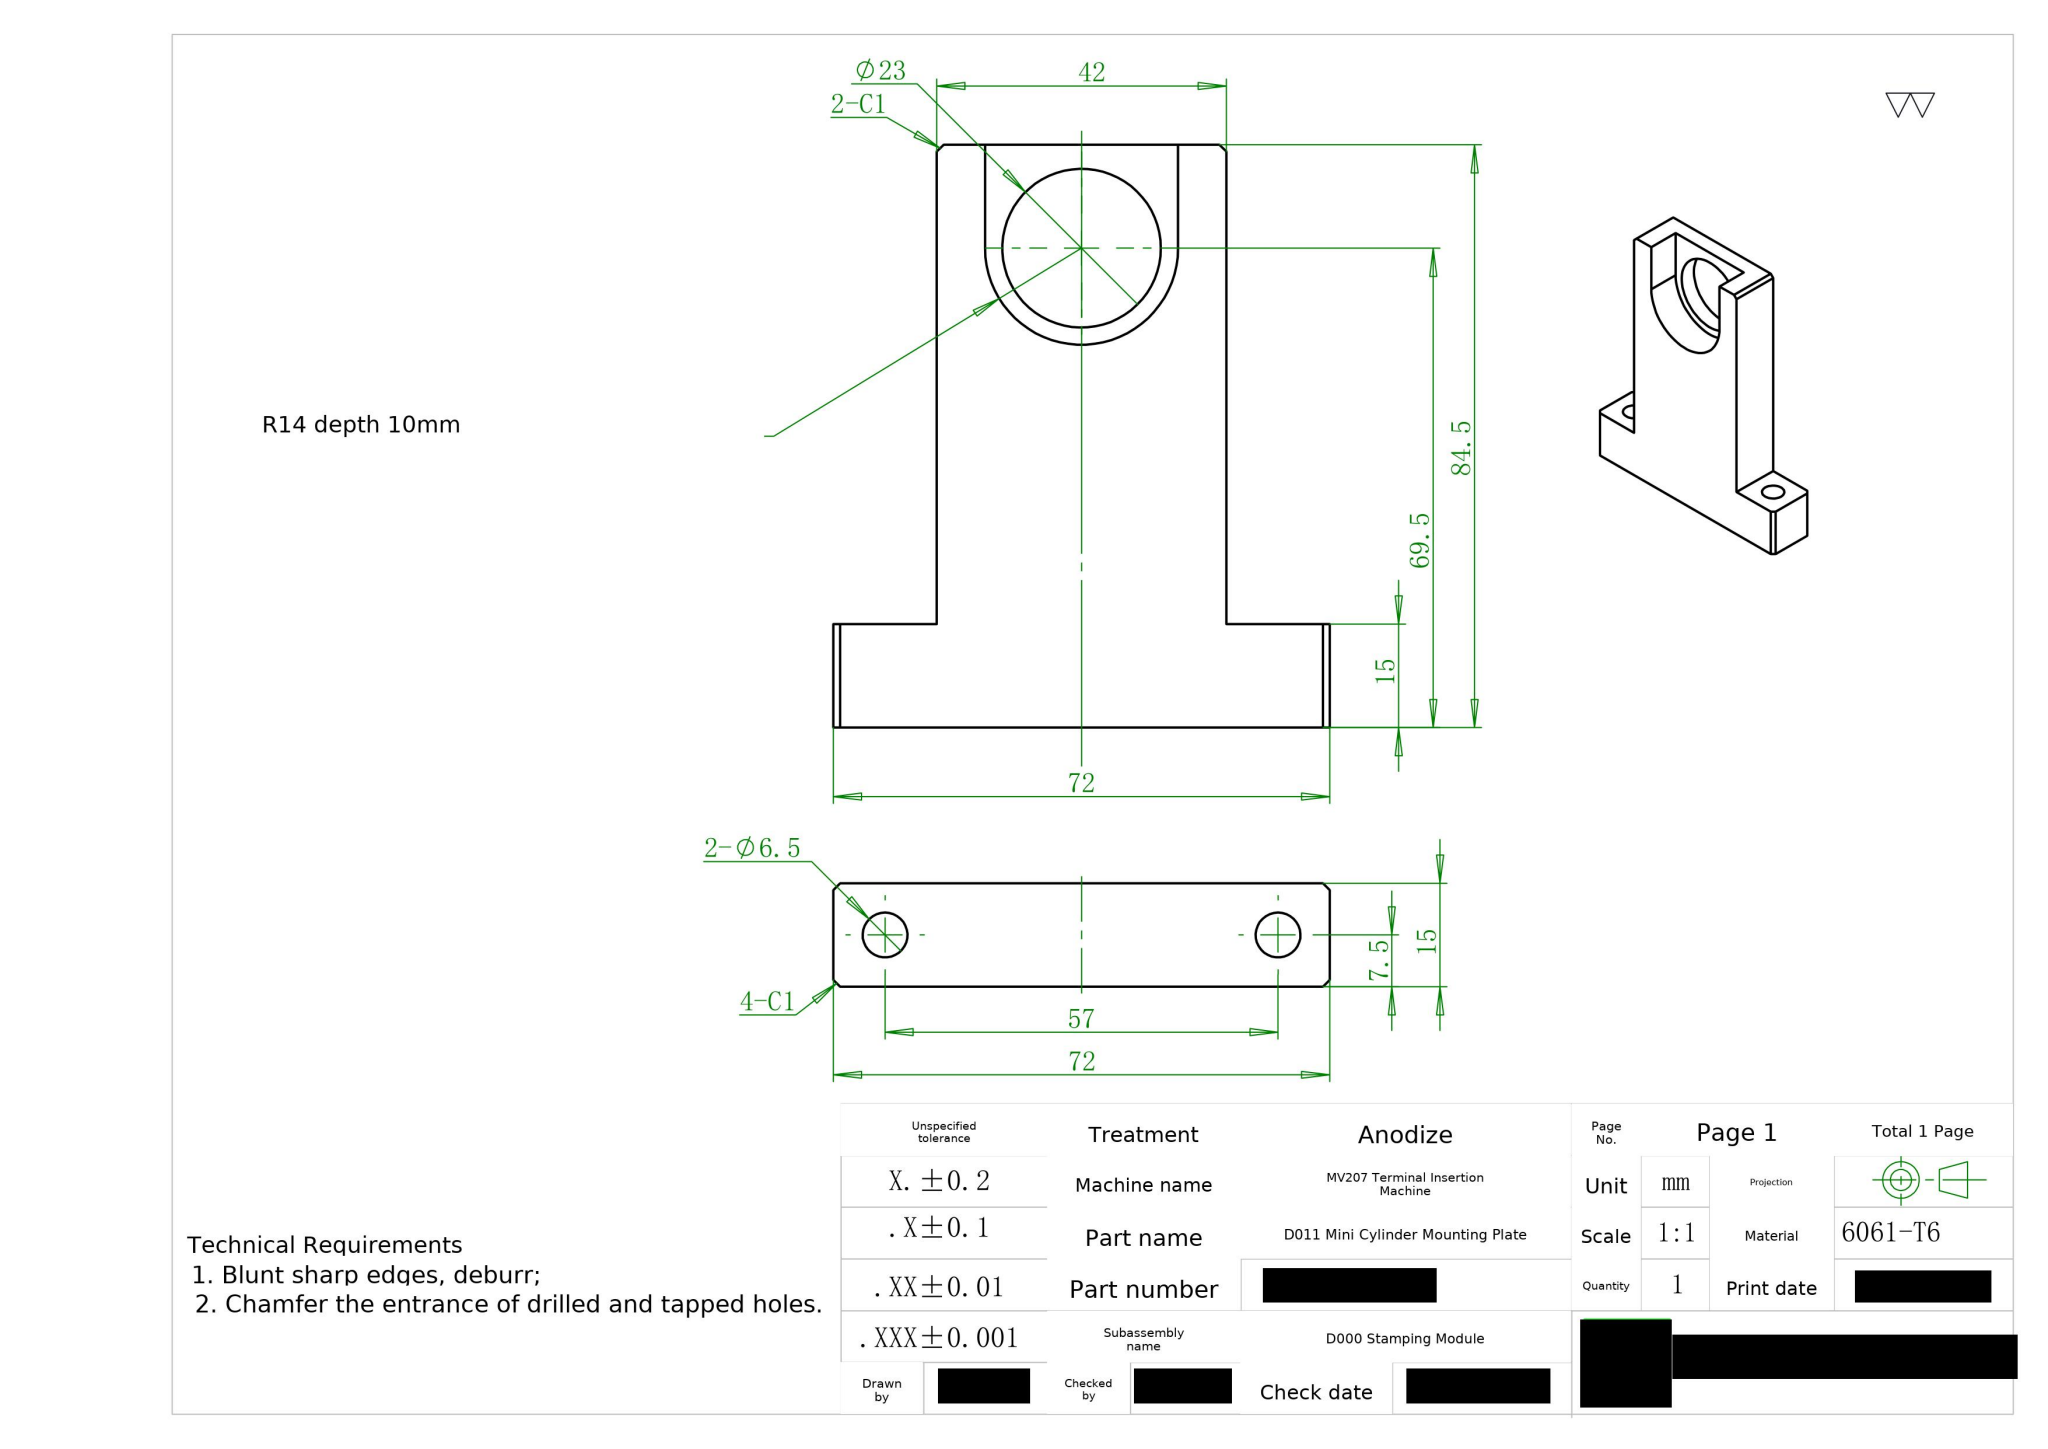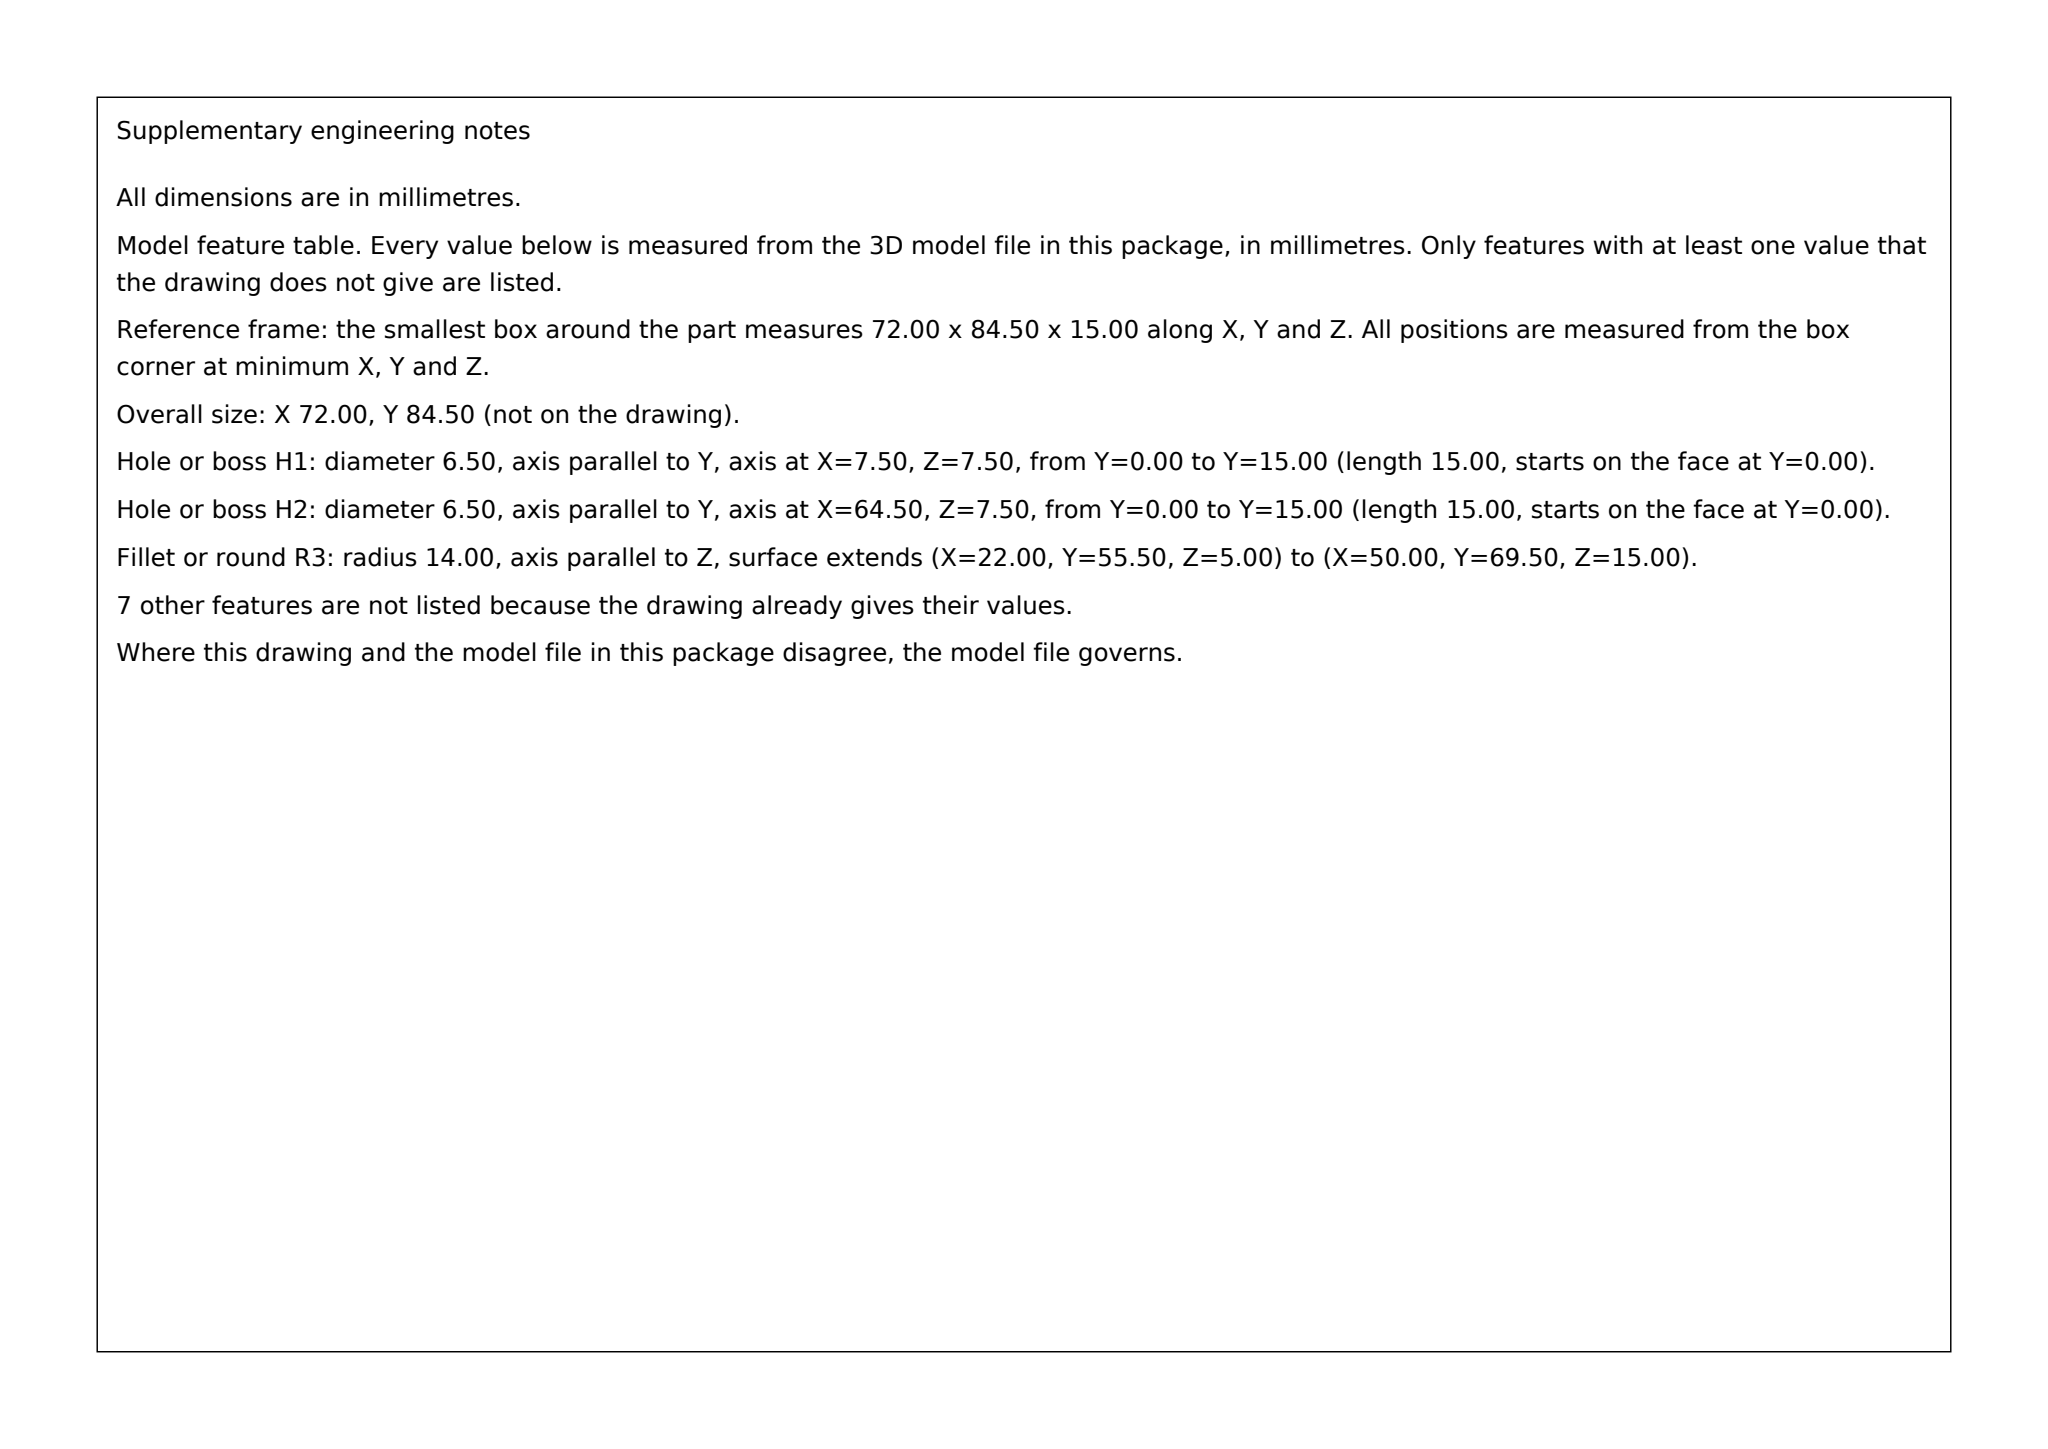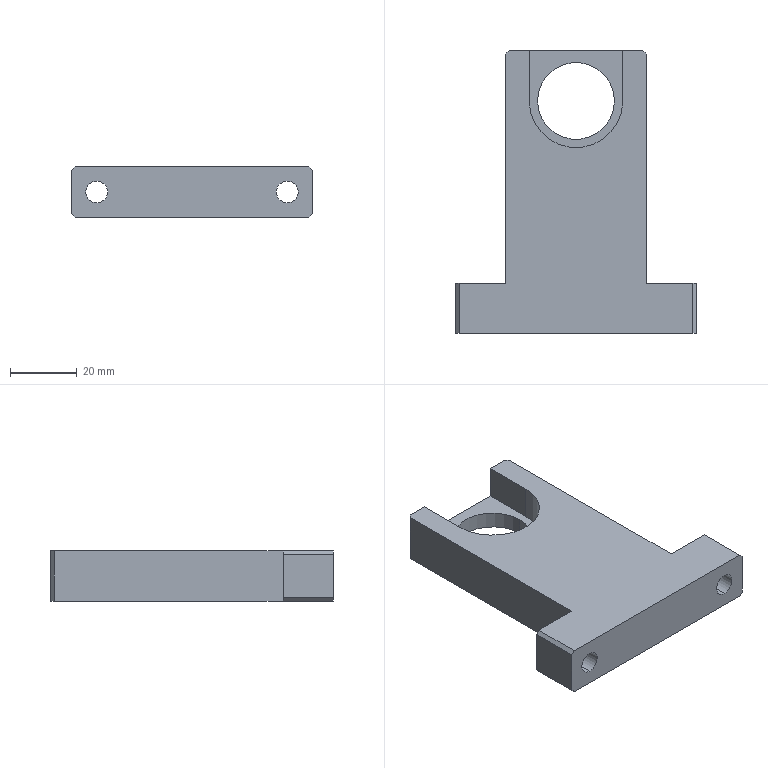Part | SolidWorks | mm | material 6061-T6 | 1 solid | 26 faces | box 72 x 84.5 x 15 mm | volume 49588 mm3 | plane 19 | cylinder 7 | commonest cylinder face diameters 6.5 x4 23 x2 28 x1
build123d program:
from build123d import *

# Parameters (mm, degrees)
SKETCH1_W                  = 42
SKETCH1_H                  = 15
BOSS_EXTRUDE1_DEPTH        = 84.5
SKETCH3_W                  = 15
SKETCH3_H                  = 15
BOSS_EXTRUDE2_DEPTH        = 15
SKETCH4_W                  = 15
SKETCH4_H                  = 15
BOSS_EXTRUDE3_DEPTH        = 15
F_6_5_6_5_DIAMETER_HOLE1_D = 6.5
CUT_EXTRUDE1_DEPTH         = 10
SKETCH11_R                 = 11.5
CUT_EXTRUDE2_DEPTH         = 93.392
CHAMFER1_SIZE              = 1


with BuildPart() as part:
    # Sketch1 → Boss-Extrude1 (new body)
    with BuildSketch(Plane(origin=(0, 0, 0), x_dir=(1, 0, 0), z_dir=(0, 1, 0))):
        Rectangle(SKETCH1_W, SKETCH1_H)
    extrude(amount=BOSS_EXTRUDE1_DEPTH)

    # Sketch3 → Boss-Extrude2 (add)
    with BuildSketch(Plane(origin=(21, 0, 0), x_dir=(0, 0, -1), z_dir=(1, 0, 0))):
        with Locations((0, 7.5)):
            Rectangle(SKETCH3_W, SKETCH3_H)
    extrude(amount=BOSS_EXTRUDE2_DEPTH)

    # Sketch4 → Boss-Extrude3 (add)
    with BuildSketch(Plane.ZY.offset(21)):
        with Locations((0, 7.5)):
            Rectangle(SKETCH4_W, SKETCH4_H)
    extrude(amount=BOSS_EXTRUDE3_DEPTH)

    # 6.5 _6.5_ Diameter Hole1 (through all)
    with Locations(Plane(origin=(0, 15, 0), x_dir=(1, 0, 0), z_dir=(0, 1, 0))):
        with Locations((-28.5, 0), (28.5, 0)):
            Hole(F_6_5_6_5_DIAMETER_HOLE1_D / 2)

    # Sketch10 → Cut-Extrude1 (cut)
    with BuildSketch(Plane.XY.offset(7.5)):
        with BuildLine():
            Line((14, 84.5), (14, 69.5))
            ThreePointArc((14, 69.5), (0, 55.5), (-14, 69.5))
            Line((-14, 69.5), (-14, 84.5))
            ThreePointArc((-14, 84.5), (0, 98.5), (14, 84.5))
        make_face()
    extrude(amount=-CUT_EXTRUDE1_DEPTH, mode=Mode.SUBTRACT)

    # Sketch11 → Cut-Extrude2 (cut, through all)
    with BuildSketch(Plane.XY.offset(-2.5)):
        with Locations((0, 69.5)):
            Circle(SKETCH11_R)
    extrude(amount=-CUT_EXTRUDE2_DEPTH, mode=Mode.SUBTRACT)

    # Chamfer1
    chamfer1_edges = [part.edges().sort_by_distance(p)[0] for p in [
        (-36, 7.5, 7.5),
        (-36, 7.5, -7.5),
        (36, 7.5, -7.5),
        (36, 7.5, 7.5),
        (21, 84.5, 0),
        (-21, 84.5, 0),
    ]]
    chamfer(chamfer1_edges, length=CHAMFER1_SIZE)


solid = part.part
STEP:
#1=CARTESIAN_POINT('',(-11.5,69.5,-7.5));
#2=VERTEX_POINT('',#1);
#3=CARTESIAN_POINT('',(11.5,69.5,-7.5));
#4=VERTEX_POINT('',#3);
#5=CARTESIAN_POINT('',(0.,69.5,-7.5));
#6=DIRECTION('',(0.,0.,1.));
#7=DIRECTION('',(1.,0.,0.));
#8=AXIS2_PLACEMENT_3D('',#5,#6,#7);
#9=CIRCLE('',#8,11.5);
#10=EDGE_CURVE('',#2,#4,#9,.T.);
#11=ORIENTED_EDGE('',*,*,#10,.F.);
#12=CARTESIAN_POINT('',(-11.5,69.5,-2.5));
#13=VERTEX_POINT('',#12);
#14=CARTESIAN_POINT('',(-11.5,69.5,-7.5));
#15=DIRECTION('',(0.,0.,1.));
#16=VECTOR('',#15,1000.);
#17=LINE('',#14,#16);
#18=EDGE_CURVE('',#2,#13,#17,.T.);
#19=ORIENTED_EDGE('',*,*,#18,.T.);
#20=CARTESIAN_POINT('',(11.5,69.5,-2.5));
#21=VERTEX_POINT('',#20);
#22=CARTESIAN_POINT('',(0.,69.5,-2.5));
#23=DIRECTION('',(0.,0.,1.));
#24=DIRECTION('',(1.,0.,0.));
#25=AXIS2_PLACEMENT_3D('',#22,#23,#24);
#26=CIRCLE('',#25,11.5);
#27=EDGE_CURVE('',#13,#21,#26,.T.);
#28=ORIENTED_EDGE('',*,*,#27,.T.);
#29=CARTESIAN_POINT('',(11.5,69.5,-7.5));
#30=DIRECTION('',(0.,0.,1.));
#31=VECTOR('',#30,1000.);
#32=LINE('',#29,#31);
#33=EDGE_CURVE('',#4,#21,#32,.T.);
#34=ORIENTED_EDGE('',*,*,#33,.F.);
#35=EDGE_LOOP('',(#11,#19,#28,#34));
#36=FACE_OUTER_BOUND('',#35,.T.);
#37=CARTESIAN_POINT('',(0.,69.5,-7.5));
#38=DIRECTION('',(0.,0.,1.));
#39=DIRECTION('',(1.,0.,0.));
#40=AXIS2_PLACEMENT_3D('',#37,#38,#39);
#41=CYLINDRICAL_SURFACE('',#40,11.5);
#42=ADVANCED_FACE('',(#36),#41,.F.);
#43=CARTESIAN_POINT('',(-28.5,0.,-3.25));
#44=VERTEX_POINT('',#43);
#45=CARTESIAN_POINT('',(-28.5,0.,3.25));
#46=VERTEX_POINT('',#45);
#47=CARTESIAN_POINT('',(-28.5,0.,0.));
#48=DIRECTION('',(0.,1.,0.));
#49=DIRECTION('',(0.,0.,1.));
#50=AXIS2_PLACEMENT_3D('',#47,#48,#49);
#51=CIRCLE('',#50,3.25);
#52=EDGE_CURVE('',#44,#46,#51,.T.);
#53=ORIENTED_EDGE('',*,*,#52,.F.);
#54=CARTESIAN_POINT('',(-28.5,15.,-3.25));
#55=VERTEX_POINT('',#54);
#56=CARTESIAN_POINT('',(-28.5,15.,-3.25));
#57=DIRECTION('',(0.,1.,0.));
#58=VECTOR('',#57,1000.);
#59=LINE('',#56,#58);
#60=EDGE_CURVE('',#44,#55,#59,.T.);
#61=ORIENTED_EDGE('',*,*,#60,.T.);
#62=CARTESIAN_POINT('',(-28.5,15.,3.25));
#63=VERTEX_POINT('',#62);
#64=CARTESIAN_POINT('',(-28.5,15.,0.));
#65=DIRECTION('',(0.,1.,0.));
#66=DIRECTION('',(0.,0.,1.));
#67=AXIS2_PLACEMENT_3D('',#64,#65,#66);
#68=CIRCLE('',#67,3.25);
#69=EDGE_CURVE('',#55,#63,#68,.T.);
#70=ORIENTED_EDGE('',*,*,#69,.T.);
#71=CARTESIAN_POINT('',(-28.5,15.,3.25));
#72=DIRECTION('',(0.,1.,0.));
#73=VECTOR('',#72,1000.);
#74=LINE('',#71,#73);
#75=EDGE_CURVE('',#46,#63,#74,.T.);
#76=ORIENTED_EDGE('',*,*,#75,.F.);
#77=EDGE_LOOP('',(#53,#61,#70,#76));
#78=FACE_OUTER_BOUND('',#77,.T.);
#79=CARTESIAN_POINT('',(-28.5,15.,0.));
#80=DIRECTION('',(0.,1.,0.));
#81=DIRECTION('',(0.,0.,1.));
#82=AXIS2_PLACEMENT_3D('',#79,#80,#81);
#83=CYLINDRICAL_SURFACE('',#82,3.25);
#84=ADVANCED_FACE('',(#78),#83,.F.);
#85=CARTESIAN_POINT('',(28.5,0.,-3.25));
#86=VERTEX_POINT('',#85);
#87=CARTESIAN_POINT('',(28.5,0.,3.25));
#88=VERTEX_POINT('',#87);
#89=CARTESIAN_POINT('',(28.5,0.,0.));
#90=DIRECTION('',(0.,1.,0.));
#91=DIRECTION('',(0.,0.,1.));
#92=AXIS2_PLACEMENT_3D('',#89,#90,#91);
#93=CIRCLE('',#92,3.25);
#94=EDGE_CURVE('',#86,#88,#93,.T.);
#95=ORIENTED_EDGE('',*,*,#94,.F.);
#96=CARTESIAN_POINT('',(28.5,15.,-3.25));
#97=VERTEX_POINT('',#96);
#98=CARTESIAN_POINT('',(28.5,15.,-3.25));
#99=DIRECTION('',(0.,1.,0.));
#100=VECTOR('',#99,1000.);
#101=LINE('',#98,#100);
#102=EDGE_CURVE('',#86,#97,#101,.T.);
#103=ORIENTED_EDGE('',*,*,#102,.T.);
#104=CARTESIAN_POINT('',(28.5,15.,3.25));
#105=VERTEX_POINT('',#104);
#106=CARTESIAN_POINT('',(28.5,15.,0.));
#107=DIRECTION('',(0.,1.,0.));
#108=DIRECTION('',(0.,0.,1.));
#109=AXIS2_PLACEMENT_3D('',#106,#107,#108);
#110=CIRCLE('',#109,3.25);
#111=EDGE_CURVE('',#97,#105,#110,.T.);
#112=ORIENTED_EDGE('',*,*,#111,.T.);
#113=CARTESIAN_POINT('',(28.5,15.,3.25));
#114=DIRECTION('',(0.,1.,0.));
#115=VECTOR('',#114,1000.);
#116=LINE('',#113,#115);
#117=EDGE_CURVE('',#88,#105,#116,.T.);
#118=ORIENTED_EDGE('',*,*,#117,.F.);
#119=EDGE_LOOP('',(#95,#103,#112,#118));
#120=FACE_OUTER_BOUND('',#119,.T.);
#121=CARTESIAN_POINT('',(28.5,15.,0.));
#122=DIRECTION('',(0.,1.,0.));
#123=DIRECTION('',(0.,0.,1.));
#124=AXIS2_PLACEMENT_3D('',#121,#122,#123);
#125=CYLINDRICAL_SURFACE('',#124,3.25);
#126=ADVANCED_FACE('',(#120),#125,.F.);
#127=CARTESIAN_POINT('',(-21.,83.5,7.5));
#128=VERTEX_POINT('',#127);
#129=CARTESIAN_POINT('',(-21.,15.,7.5));
#130=VERTEX_POINT('',#129);
#131=CARTESIAN_POINT('',(-21.,84.5,7.5));
#132=DIRECTION('',(0.,-1.,0.));
#133=VECTOR('',#132,1000.);
#134=LINE('',#131,#133);
#135=EDGE_CURVE('',#128,#130,#134,.T.);
#136=ORIENTED_EDGE('',*,*,#135,.F.);
#137=CARTESIAN_POINT('',(-21.,83.5,-7.5));
#138=VERTEX_POINT('',#137);
#139=CARTESIAN_POINT('',(-21.,83.5,-7.5));
#140=DIRECTION('',(0.,0.,-1.));
#141=VECTOR('',#140,1000.);
#142=LINE('',#139,#141);
#143=EDGE_CURVE('',#128,#138,#142,.T.);
#144=ORIENTED_EDGE('',*,*,#143,.T.);
#145=CARTESIAN_POINT('',(-21.,15.,-7.5));
#146=VERTEX_POINT('',#145);
#147=CARTESIAN_POINT('',(-21.,84.5,-7.5));
#148=DIRECTION('',(0.,-1.,0.));
#149=VECTOR('',#148,1000.);
#150=LINE('',#147,#149);
#151=EDGE_CURVE('',#138,#146,#150,.T.);
#152=ORIENTED_EDGE('',*,*,#151,.T.);
#153=CARTESIAN_POINT('',(-21.,15.,7.5));
#154=DIRECTION('',(0.,-0.,-1.));
#155=VECTOR('',#154,1000.);
#156=LINE('',#153,#155);
#157=EDGE_CURVE('',#130,#146,#156,.T.);
#158=ORIENTED_EDGE('',*,*,#157,.F.);
#159=EDGE_LOOP('',(#136,#144,#152,#158));
#160=FACE_OUTER_BOUND('',#159,.T.);
#161=CARTESIAN_POINT('',(-21.,84.5,-7.5));
#162=DIRECTION('',(1.,0.,0.));
#163=DIRECTION('',(0.,0.,-1.));
#164=AXIS2_PLACEMENT_3D('',#161,#162,#163);
#165=PLANE('',#164);
#166=ADVANCED_FACE('',(#160),#165,.F.);
#167=CARTESIAN_POINT('',(21.,83.5,-7.5));
#168=VERTEX_POINT('',#167);
#169=CARTESIAN_POINT('',(21.,15.,-7.5));
#170=VERTEX_POINT('',#169);
#171=CARTESIAN_POINT('',(21.,84.5,-7.5));
#172=DIRECTION('',(0.,-1.,0.));
#173=VECTOR('',#172,1000.);
#174=LINE('',#171,#173);
#175=EDGE_CURVE('',#168,#170,#174,.T.);
#176=ORIENTED_EDGE('',*,*,#175,.F.);
#177=CARTESIAN_POINT('',(21.,83.5,7.5));
#178=VERTEX_POINT('',#177);
#179=CARTESIAN_POINT('',(21.,83.5,7.5));
#180=DIRECTION('',(0.,0.,1.));
#181=VECTOR('',#180,1000.);
#182=LINE('',#179,#181);
#183=EDGE_CURVE('',#168,#178,#182,.T.);
#184=ORIENTED_EDGE('',*,*,#183,.T.);
#185=CARTESIAN_POINT('',(21.,15.,7.5));
#186=VERTEX_POINT('',#185);
#187=CARTESIAN_POINT('',(21.,84.5,7.5));
#188=DIRECTION('',(0.,-1.,0.));
#189=VECTOR('',#188,1000.);
#190=LINE('',#187,#189);
#191=EDGE_CURVE('',#178,#186,#190,.T.);
#192=ORIENTED_EDGE('',*,*,#191,.T.);
#193=CARTESIAN_POINT('',(21.,15.,7.5));
#194=DIRECTION('',(0.,0.,1.));
#195=VECTOR('',#194,1000.);
#196=LINE('',#193,#195);
#197=EDGE_CURVE('',#170,#186,#196,.T.);
#198=ORIENTED_EDGE('',*,*,#197,.F.);
#199=EDGE_LOOP('',(#176,#184,#192,#198));
#200=FACE_OUTER_BOUND('',#199,.T.);
#201=CARTESIAN_POINT('',(21.,84.5,-7.5));
#202=DIRECTION('',(-1.,0.,0.));
#203=DIRECTION('',(0.,0.,1.));
#204=AXIS2_PLACEMENT_3D('',#201,#202,#203);
#205=PLANE('',#204);
#206=ADVANCED_FACE('',(#200),#205,.F.);
#207=CARTESIAN_POINT('',(0.,69.5,-7.5));
#208=DIRECTION('',(0.,0.,1.));
#209=DIRECTION('',(1.,0.,0.));
#210=AXIS2_PLACEMENT_3D('',#207,#208,#209);
#211=CIRCLE('',#210,11.5);
#212=EDGE_CURVE('',#4,#2,#211,.T.);
#213=ORIENTED_EDGE('',*,*,#212,.T.);
#214=ORIENTED_EDGE('',*,*,#10,.T.);
#215=EDGE_LOOP('',(#213,#214));
#216=FACE_BOUND('',#215,.T.);
#217=CARTESIAN_POINT('',(35.,0.,-7.5));
#218=VERTEX_POINT('',#217);
#219=CARTESIAN_POINT('',(-35.,0.,-7.5));
#220=VERTEX_POINT('',#219);
#221=CARTESIAN_POINT('',(-21.,0.,-7.5));
#222=DIRECTION('',(-1.,0.,0.));
#223=VECTOR('',#222,1000.);
#224=LINE('',#221,#223);
#225=EDGE_CURVE('',#218,#220,#224,.T.);
#226=ORIENTED_EDGE('',*,*,#225,.T.);
#227=CARTESIAN_POINT('',(-35.,15.,-7.5));
#228=VERTEX_POINT('',#227);
#229=CARTESIAN_POINT('',(-35.,15.,-7.5));
#230=DIRECTION('',(0.,1.,0.));
#231=VECTOR('',#230,1000.);
#232=LINE('',#229,#231);
#233=EDGE_CURVE('',#220,#228,#232,.T.);
#234=ORIENTED_EDGE('',*,*,#233,.T.);
#235=CARTESIAN_POINT('',(-36.,15.,-7.5));
#236=DIRECTION('',(1.,0.,0.));
#237=VECTOR('',#236,1000.);
#238=LINE('',#235,#237);
#239=EDGE_CURVE('',#228,#146,#238,.T.);
#240=ORIENTED_EDGE('',*,*,#239,.T.);
#241=ORIENTED_EDGE('',*,*,#151,.F.);
#242=CARTESIAN_POINT('',(-20.,84.5,-7.5));
#243=VERTEX_POINT('',#242);
#244=CARTESIAN_POINT('',(-20.,84.5,-7.5));
#245=DIRECTION('',(0.7071,0.7071,0.));
#246=VECTOR('',#245,1000.);
#247=LINE('',#244,#246);
#248=EDGE_CURVE('',#138,#243,#247,.T.);
#249=ORIENTED_EDGE('',*,*,#248,.T.);
#250=CARTESIAN_POINT('',(20.,84.5,-7.5));
#251=VERTEX_POINT('',#250);
#252=CARTESIAN_POINT('',(-21.,84.5,-7.5));
#253=DIRECTION('',(-1.,0.,0.));
#254=VECTOR('',#253,1000.);
#255=LINE('',#252,#254);
#256=EDGE_CURVE('',#251,#243,#255,.T.);
#257=ORIENTED_EDGE('',*,*,#256,.F.);
#258=CARTESIAN_POINT('',(20.,84.5,-7.5));
#259=DIRECTION('',(0.7071,-0.7071,0.));
#260=VECTOR('',#259,1000.);
#261=LINE('',#258,#260);
#262=EDGE_CURVE('',#251,#168,#261,.T.);
#263=ORIENTED_EDGE('',*,*,#262,.T.);
#264=ORIENTED_EDGE('',*,*,#175,.T.);
#265=CARTESIAN_POINT('',(35.,15.,-7.5));
#266=VERTEX_POINT('',#265);
#267=CARTESIAN_POINT('',(36.,15.,-7.5));
#268=DIRECTION('',(-1.,0.,0.));
#269=VECTOR('',#268,1000.);
#270=LINE('',#267,#269);
#271=EDGE_CURVE('',#266,#170,#270,.T.);
#272=ORIENTED_EDGE('',*,*,#271,.F.);
#273=CARTESIAN_POINT('',(35.,84.5,-7.5));
#274=DIRECTION('',(0.,-1.,0.));
#275=VECTOR('',#274,1000.);
#276=LINE('',#273,#275);
#277=EDGE_CURVE('',#266,#218,#276,.T.);
#278=ORIENTED_EDGE('',*,*,#277,.T.);
#279=EDGE_LOOP('',(#226,#234,#240,#241,#249,#257,#263,#264,#272,#278));
#280=FACE_OUTER_BOUND('',#279,.T.);
#281=CARTESIAN_POINT('',(-21.,84.5,-7.5));
#282=DIRECTION('',(0.,0.,1.));
#283=DIRECTION('',(1.,0.,0.));
#284=AXIS2_PLACEMENT_3D('',#281,#282,#283);
#285=PLANE('',#284);
#286=ADVANCED_FACE('',(#216,#280),#285,.F.);
#287=CARTESIAN_POINT('',(-35.,15.,7.5));
#288=VERTEX_POINT('',#287);
#289=CARTESIAN_POINT('',(-36.,15.,7.5));
#290=DIRECTION('',(1.,0.,0.));
#291=VECTOR('',#290,1000.);
#292=LINE('',#289,#291);
#293=EDGE_CURVE('',#288,#130,#292,.T.);
#294=ORIENTED_EDGE('',*,*,#293,.F.);
#295=CARTESIAN_POINT('',(-35.,0.,7.5));
#296=VERTEX_POINT('',#295);
#297=CARTESIAN_POINT('',(-35.,0.,7.5));
#298=DIRECTION('',(0.,-1.,0.));
#299=VECTOR('',#298,1000.);
#300=LINE('',#297,#299);
#301=EDGE_CURVE('',#288,#296,#300,.T.);
#302=ORIENTED_EDGE('',*,*,#301,.T.);
#303=CARTESIAN_POINT('',(35.,0.,7.5));
#304=VERTEX_POINT('',#303);
#305=CARTESIAN_POINT('',(-21.,0.,7.5));
#306=DIRECTION('',(1.,0.,0.));
#307=VECTOR('',#306,1000.);
#308=LINE('',#305,#307);
#309=EDGE_CURVE('',#296,#304,#308,.T.);
#310=ORIENTED_EDGE('',*,*,#309,.T.);
#311=CARTESIAN_POINT('',(35.,15.,7.5));
#312=VERTEX_POINT('',#311);
#313=CARTESIAN_POINT('',(35.,84.5,7.5));
#314=DIRECTION('',(0.,1.,0.));
#315=VECTOR('',#314,1000.);
#316=LINE('',#313,#315);
#317=EDGE_CURVE('',#304,#312,#316,.T.);
#318=ORIENTED_EDGE('',*,*,#317,.T.);
#319=CARTESIAN_POINT('',(36.,15.,7.5));
#320=DIRECTION('',(-1.,0.,0.));
#321=VECTOR('',#320,1000.);
#322=LINE('',#319,#321);
#323=EDGE_CURVE('',#312,#186,#322,.T.);
#324=ORIENTED_EDGE('',*,*,#323,.T.);
#325=ORIENTED_EDGE('',*,*,#191,.F.);
#326=CARTESIAN_POINT('',(20.,84.5,7.5));
#327=VERTEX_POINT('',#326);
#328=CARTESIAN_POINT('',(20.,84.5,7.5));
#329=DIRECTION('',(-0.7071,0.7071,0.));
#330=VECTOR('',#329,1000.);
#331=LINE('',#328,#330);
#332=EDGE_CURVE('',#178,#327,#331,.T.);
#333=ORIENTED_EDGE('',*,*,#332,.T.);
#334=CARTESIAN_POINT('',(14.,84.5,7.5));
#335=VERTEX_POINT('',#334);
#336=CARTESIAN_POINT('',(-21.,84.5,7.5));
#337=DIRECTION('',(1.,0.,0.));
#338=VECTOR('',#337,1000.);
#339=LINE('',#336,#338);
#340=EDGE_CURVE('',#335,#327,#339,.T.);
#341=ORIENTED_EDGE('',*,*,#340,.F.);
#342=CARTESIAN_POINT('',(14.,69.5,7.5));
#343=VERTEX_POINT('',#342);
#344=CARTESIAN_POINT('',(14.,84.5,7.5));
#345=DIRECTION('',(0.,1.,0.));
#346=VECTOR('',#345,1000.);
#347=LINE('',#344,#346);
#348=EDGE_CURVE('',#343,#335,#347,.T.);
#349=ORIENTED_EDGE('',*,*,#348,.F.);
#350=CARTESIAN_POINT('',(-14.,69.5,7.5));
#351=VERTEX_POINT('',#350);
#352=CARTESIAN_POINT('',(0.,69.5,7.5));
#353=DIRECTION('',(0.,0.,1.));
#354=DIRECTION('',(1.,0.,0.));
#355=AXIS2_PLACEMENT_3D('',#352,#353,#354);
#356=CIRCLE('',#355,14.);
#357=EDGE_CURVE('',#351,#343,#356,.T.);
#358=ORIENTED_EDGE('',*,*,#357,.F.);
#359=CARTESIAN_POINT('',(-14.,84.5,7.5));
#360=VERTEX_POINT('',#359);
#361=CARTESIAN_POINT('',(-14.,84.5,7.5));
#362=DIRECTION('',(0.,-1.,0.));
#363=VECTOR('',#362,1000.);
#364=LINE('',#361,#363);
#365=EDGE_CURVE('',#360,#351,#364,.T.);
#366=ORIENTED_EDGE('',*,*,#365,.F.);
#367=CARTESIAN_POINT('',(-20.,84.5,7.5));
#368=VERTEX_POINT('',#367);
#369=CARTESIAN_POINT('',(-21.,84.5,7.5));
#370=DIRECTION('',(1.,0.,0.));
#371=VECTOR('',#370,1000.);
#372=LINE('',#369,#371);
#373=EDGE_CURVE('',#368,#360,#372,.T.);
#374=ORIENTED_EDGE('',*,*,#373,.F.);
#375=CARTESIAN_POINT('',(-20.,84.5,7.5));
#376=DIRECTION('',(-0.7071,-0.7071,0.));
#377=VECTOR('',#376,1000.);
#378=LINE('',#375,#377);
#379=EDGE_CURVE('',#368,#128,#378,.T.);
#380=ORIENTED_EDGE('',*,*,#379,.T.);
#381=ORIENTED_EDGE('',*,*,#135,.T.);
#382=EDGE_LOOP('',(#294,#302,#310,#318,#324,#325,#333,#341,#349,#358,#366,#374,#380,#381));
#383=FACE_OUTER_BOUND('',#382,.T.);
#384=CARTESIAN_POINT('',(-21.,84.5,7.5));
#385=DIRECTION('',(0.,0.,-1.));
#386=DIRECTION('',(-1.,0.,0.));
#387=AXIS2_PLACEMENT_3D('',#384,#385,#386);
#388=PLANE('',#387);
#389=ADVANCED_FACE('',(#383),#388,.F.);
#390=ORIENTED_EDGE('',*,*,#340,.T.);
#391=CARTESIAN_POINT('',(20.,84.5,-7.5));
#392=DIRECTION('',(0.,0.,-1.));
#393=VECTOR('',#392,1000.);
#394=LINE('',#391,#393);
#395=EDGE_CURVE('',#327,#251,#394,.T.);
#396=ORIENTED_EDGE('',*,*,#395,.T.);
#397=ORIENTED_EDGE('',*,*,#256,.T.);
#398=CARTESIAN_POINT('',(-20.,84.5,7.5));
#399=DIRECTION('',(0.,0.,1.));
#400=VECTOR('',#399,1000.);
#401=LINE('',#398,#400);
#402=EDGE_CURVE('',#243,#368,#401,.T.);
#403=ORIENTED_EDGE('',*,*,#402,.T.);
#404=ORIENTED_EDGE('',*,*,#373,.T.);
#405=CARTESIAN_POINT('',(-14.,84.5,-2.5));
#406=VERTEX_POINT('',#405);
#407=CARTESIAN_POINT('',(-14.,84.5,-2.5));
#408=DIRECTION('',(0.,0.,1.));
#409=VECTOR('',#408,1000.);
#410=LINE('',#407,#409);
#411=EDGE_CURVE('',#406,#360,#410,.T.);
#412=ORIENTED_EDGE('',*,*,#411,.F.);
#413=CARTESIAN_POINT('',(14.,84.5,-2.5));
#414=VERTEX_POINT('',#413);
#415=CARTESIAN_POINT('',(0.,84.5,-2.5));
#416=DIRECTION('',(1.,0.,0.));
#417=VECTOR('',#416,1000.);
#418=LINE('',#415,#417);
#419=EDGE_CURVE('',#406,#414,#418,.T.);
#420=ORIENTED_EDGE('',*,*,#419,.T.);
#421=CARTESIAN_POINT('',(14.,84.5,-2.5));
#422=DIRECTION('',(0.,0.,1.));
#423=VECTOR('',#422,1000.);
#424=LINE('',#421,#423);
#425=EDGE_CURVE('',#414,#335,#424,.T.);
#426=ORIENTED_EDGE('',*,*,#425,.T.);
#427=EDGE_LOOP('',(#390,#396,#397,#403,#404,#412,#420,#426));
#428=FACE_OUTER_BOUND('',#427,.T.);
#429=CARTESIAN_POINT('',(0.,84.5,0.));
#430=DIRECTION('',(0.,1.,0.));
#431=DIRECTION('',(0.,0.,1.));
#432=AXIS2_PLACEMENT_3D('',#429,#430,#431);
#433=PLANE('',#432);
#434=ADVANCED_FACE('',(#428),#433,.T.);
#435=CARTESIAN_POINT('',(-28.5,0.,0.));
#436=DIRECTION('',(0.,1.,0.));
#437=DIRECTION('',(0.,0.,1.));
#438=AXIS2_PLACEMENT_3D('',#435,#436,#437);
#439=CIRCLE('',#438,3.25);
#440=EDGE_CURVE('',#46,#44,#439,.T.);
#441=ORIENTED_EDGE('',*,*,#440,.T.);
#442=ORIENTED_EDGE('',*,*,#52,.T.);
#443=EDGE_LOOP('',(#441,#442));
#444=FACE_BOUND('',#443,.T.);
#445=CARTESIAN_POINT('',(28.5,0.,0.));
#446=DIRECTION('',(0.,1.,0.));
#447=DIRECTION('',(0.,0.,1.));
#448=AXIS2_PLACEMENT_3D('',#445,#446,#447);
#449=CIRCLE('',#448,3.25);
#450=EDGE_CURVE('',#88,#86,#449,.T.);
#451=ORIENTED_EDGE('',*,*,#450,.T.);
#452=ORIENTED_EDGE('',*,*,#94,.T.);
#453=EDGE_LOOP('',(#451,#452));
#454=FACE_BOUND('',#453,.T.);
#455=ORIENTED_EDGE('',*,*,#309,.F.);
#456=CARTESIAN_POINT('',(-36.,-0.,6.5));
#457=VERTEX_POINT('',#456);
#458=CARTESIAN_POINT('',(-36.,0.,6.5));
#459=DIRECTION('',(-0.7071,0.,-0.7071));
#460=VECTOR('',#459,1000.);
#461=LINE('',#458,#460);
#462=EDGE_CURVE('',#296,#457,#461,.T.);
#463=ORIENTED_EDGE('',*,*,#462,.T.);
#464=CARTESIAN_POINT('',(-36.,-0.,-6.5));
#465=VERTEX_POINT('',#464);
#466=CARTESIAN_POINT('',(-36.,0.,7.5));
#467=DIRECTION('',(0.,0.,1.));
#468=VECTOR('',#467,1000.);
#469=LINE('',#466,#468);
#470=EDGE_CURVE('',#465,#457,#469,.T.);
#471=ORIENTED_EDGE('',*,*,#470,.F.);
#472=CARTESIAN_POINT('',(-36.,0.,-6.5));
#473=DIRECTION('',(0.7071,0.,-0.7071));
#474=VECTOR('',#473,1000.);
#475=LINE('',#472,#474);
#476=EDGE_CURVE('',#465,#220,#475,.T.);
#477=ORIENTED_EDGE('',*,*,#476,.T.);
#478=ORIENTED_EDGE('',*,*,#225,.F.);
#479=CARTESIAN_POINT('',(36.,0.,-6.5));
#480=VERTEX_POINT('',#479);
#481=CARTESIAN_POINT('',(36.,0.,-6.5));
#482=DIRECTION('',(0.7071,0.,0.7071));
#483=VECTOR('',#482,1000.);
#484=LINE('',#481,#483);
#485=EDGE_CURVE('',#218,#480,#484,.T.);
#486=ORIENTED_EDGE('',*,*,#485,.T.);
#487=CARTESIAN_POINT('',(36.,0.,6.5));
#488=VERTEX_POINT('',#487);
#489=CARTESIAN_POINT('',(36.,0.,7.5));
#490=DIRECTION('',(0.,0.,-1.));
#491=VECTOR('',#490,1000.);
#492=LINE('',#489,#491);
#493=EDGE_CURVE('',#488,#480,#492,.T.);
#494=ORIENTED_EDGE('',*,*,#493,.F.);
#495=CARTESIAN_POINT('',(36.,0.,6.5));
#496=DIRECTION('',(-0.7071,0.,0.7071));
#497=VECTOR('',#496,1000.);
#498=LINE('',#495,#497);
#499=EDGE_CURVE('',#488,#304,#498,.T.);
#500=ORIENTED_EDGE('',*,*,#499,.T.);
#501=EDGE_LOOP('',(#455,#463,#471,#477,#478,#486,#494,#500));
#502=FACE_OUTER_BOUND('',#501,.T.);
#503=CARTESIAN_POINT('',(0.,0.,0.));
#504=DIRECTION('',(0.,1.,0.));
#505=DIRECTION('',(0.,0.,1.));
#506=AXIS2_PLACEMENT_3D('',#503,#504,#505);
#507=PLANE('',#506);
#508=ADVANCED_FACE('',(#444,#454,#502),#507,.F.);
#509=CARTESIAN_POINT('',(28.5,15.,0.));
#510=DIRECTION('',(0.,1.,0.));
#511=DIRECTION('',(0.,0.,1.));
#512=AXIS2_PLACEMENT_3D('',#509,#510,#511);
#513=CIRCLE('',#512,3.25);
#514=EDGE_CURVE('',#105,#97,#513,.T.);
#515=ORIENTED_EDGE('',*,*,#514,.F.);
#516=ORIENTED_EDGE('',*,*,#111,.F.);
#517=EDGE_LOOP('',(#515,#516));
#518=FACE_BOUND('',#517,.T.);
#519=CARTESIAN_POINT('',(36.,15.,-6.5));
#520=VERTEX_POINT('',#519);
#521=CARTESIAN_POINT('',(36.,15.,6.5));
#522=VERTEX_POINT('',#521);
#523=CARTESIAN_POINT('',(36.,15.,7.5));
#524=DIRECTION('',(0.,0.,1.));
#525=VECTOR('',#524,1000.);
#526=LINE('',#523,#525);
#527=EDGE_CURVE('',#520,#522,#526,.T.);
#528=ORIENTED_EDGE('',*,*,#527,.F.);
#529=CARTESIAN_POINT('',(36.,15.,-6.5));
#530=DIRECTION('',(-0.7071,0.,-0.7071));
#531=VECTOR('',#530,1000.);
#532=LINE('',#529,#531);
#533=EDGE_CURVE('',#520,#266,#532,.T.);
#534=ORIENTED_EDGE('',*,*,#533,.T.);
#535=ORIENTED_EDGE('',*,*,#271,.T.);
#536=ORIENTED_EDGE('',*,*,#197,.T.);
#537=ORIENTED_EDGE('',*,*,#323,.F.);
#538=CARTESIAN_POINT('',(36.,15.,6.5));
#539=DIRECTION('',(0.7071,0.,-0.7071));
#540=VECTOR('',#539,1000.);
#541=LINE('',#538,#540);
#542=EDGE_CURVE('',#312,#522,#541,.T.);
#543=ORIENTED_EDGE('',*,*,#542,.T.);
#544=EDGE_LOOP('',(#528,#534,#535,#536,#537,#543));
#545=FACE_OUTER_BOUND('',#544,.T.);
#546=CARTESIAN_POINT('',(36.,15.,7.5));
#547=DIRECTION('',(0.,-1.,0.));
#548=DIRECTION('',(0.,0.,-1.));
#549=AXIS2_PLACEMENT_3D('',#546,#547,#548);
#550=PLANE('',#549);
#551=ADVANCED_FACE('',(#518,#545),#550,.F.);
#552=ORIENTED_EDGE('',*,*,#493,.T.);
#553=CARTESIAN_POINT('',(36.,0.,-6.5));
#554=DIRECTION('',(0.,1.,0.));
#555=VECTOR('',#554,1000.);
#556=LINE('',#553,#555);
#557=EDGE_CURVE('',#480,#520,#556,.T.);
#558=ORIENTED_EDGE('',*,*,#557,.T.);
#559=ORIENTED_EDGE('',*,*,#527,.T.);
#560=CARTESIAN_POINT('',(36.,0.,6.5));
#561=DIRECTION('',(0.,-1.,0.));
#562=VECTOR('',#561,1000.);
#563=LINE('',#560,#562);
#564=EDGE_CURVE('',#522,#488,#563,.T.);
#565=ORIENTED_EDGE('',*,*,#564,.T.);
#566=EDGE_LOOP('',(#552,#558,#559,#565));
#567=FACE_OUTER_BOUND('',#566,.T.);
#568=CARTESIAN_POINT('',(36.,0.,0.));
#569=DIRECTION('',(-1.,0.,0.));
#570=DIRECTION('',(0.,0.,1.));
#571=AXIS2_PLACEMENT_3D('',#568,#569,#570);
#572=PLANE('',#571);
#573=ADVANCED_FACE('',(#567),#572,.F.);
#574=CARTESIAN_POINT('',(-28.5,15.,0.));
#575=DIRECTION('',(0.,1.,0.));
#576=DIRECTION('',(0.,0.,1.));
#577=AXIS2_PLACEMENT_3D('',#574,#575,#576);
#578=CIRCLE('',#577,3.25);
#579=EDGE_CURVE('',#63,#55,#578,.T.);
#580=ORIENTED_EDGE('',*,*,#579,.F.);
#581=ORIENTED_EDGE('',*,*,#69,.F.);
#582=EDGE_LOOP('',(#580,#581));
#583=FACE_BOUND('',#582,.T.);
#584=CARTESIAN_POINT('',(-36.,15.,6.5));
#585=VERTEX_POINT('',#584);
#586=CARTESIAN_POINT('',(-36.,15.,-6.5));
#587=VERTEX_POINT('',#586);
#588=CARTESIAN_POINT('',(-36.,15.,7.5));
#589=DIRECTION('',(0.,-0.,-1.));
#590=VECTOR('',#589,1000.);
#591=LINE('',#588,#590);
#592=EDGE_CURVE('',#585,#587,#591,.T.);
#593=ORIENTED_EDGE('',*,*,#592,.F.);
#594=CARTESIAN_POINT('',(-36.,15.,6.5));
#595=DIRECTION('',(0.7071,0.,0.7071));
#596=VECTOR('',#595,1000.);
#597=LINE('',#594,#596);
#598=EDGE_CURVE('',#585,#288,#597,.T.);
#599=ORIENTED_EDGE('',*,*,#598,.T.);
#600=ORIENTED_EDGE('',*,*,#293,.T.);
#601=ORIENTED_EDGE('',*,*,#157,.T.);
#602=ORIENTED_EDGE('',*,*,#239,.F.);
#603=CARTESIAN_POINT('',(-36.,15.,-6.5));
#604=DIRECTION('',(-0.7071,0.,0.7071));
#605=VECTOR('',#604,1000.);
#606=LINE('',#603,#605);
#607=EDGE_CURVE('',#228,#587,#606,.T.);
#608=ORIENTED_EDGE('',*,*,#607,.T.);
#609=EDGE_LOOP('',(#593,#599,#600,#601,#602,#608));
#610=FACE_OUTER_BOUND('',#609,.T.);
#611=CARTESIAN_POINT('',(-36.,15.,7.5));
#612=DIRECTION('',(0.,-1.,0.));
#613=DIRECTION('',(0.,-0.,-1.));
#614=AXIS2_PLACEMENT_3D('',#611,#612,#613);
#615=PLANE('',#614);
#616=ADVANCED_FACE('',(#583,#610),#615,.F.);
#617=ORIENTED_EDGE('',*,*,#470,.T.);
#618=CARTESIAN_POINT('',(-36.,15.,6.5));
#619=DIRECTION('',(0.,1.,0.));
#620=VECTOR('',#619,1000.);
#621=LINE('',#618,#620);
#622=EDGE_CURVE('',#457,#585,#621,.T.);
#623=ORIENTED_EDGE('',*,*,#622,.T.);
#624=ORIENTED_EDGE('',*,*,#592,.T.);
#625=CARTESIAN_POINT('',(-36.,-0.,-6.5));
#626=DIRECTION('',(0.,-1.,0.));
#627=VECTOR('',#626,1000.);
#628=LINE('',#625,#627);
#629=EDGE_CURVE('',#587,#465,#628,.T.);
#630=ORIENTED_EDGE('',*,*,#629,.T.);
#631=EDGE_LOOP('',(#617,#623,#624,#630));
#632=FACE_OUTER_BOUND('',#631,.T.);
#633=CARTESIAN_POINT('',(-36.,0.,0.));
#634=DIRECTION('',(-1.,0.,0.));
#635=DIRECTION('',(0.,0.,1.));
#636=AXIS2_PLACEMENT_3D('',#633,#634,#635);
#637=PLANE('',#636);
#638=ADVANCED_FACE('',(#632),#637,.T.);
#639=ORIENTED_EDGE('',*,*,#102,.F.);
#640=ORIENTED_EDGE('',*,*,#450,.F.);
#641=ORIENTED_EDGE('',*,*,#117,.T.);
#642=ORIENTED_EDGE('',*,*,#514,.T.);
#643=EDGE_LOOP('',(#639,#640,#641,#642));
#644=FACE_OUTER_BOUND('',#643,.T.);
#645=CARTESIAN_POINT('',(28.5,15.,0.));
#646=DIRECTION('',(0.,1.,0.));
#647=DIRECTION('',(0.,0.,1.));
#648=AXIS2_PLACEMENT_3D('',#645,#646,#647);
#649=CYLINDRICAL_SURFACE('',#648,3.25);
#650=ADVANCED_FACE('',(#644),#649,.F.);
#651=ORIENTED_EDGE('',*,*,#60,.F.);
#652=ORIENTED_EDGE('',*,*,#440,.F.);
#653=ORIENTED_EDGE('',*,*,#75,.T.);
#654=ORIENTED_EDGE('',*,*,#579,.T.);
#655=EDGE_LOOP('',(#651,#652,#653,#654));
#656=FACE_OUTER_BOUND('',#655,.T.);
#657=CARTESIAN_POINT('',(-28.5,15.,0.));
#658=DIRECTION('',(0.,1.,0.));
#659=DIRECTION('',(0.,0.,1.));
#660=AXIS2_PLACEMENT_3D('',#657,#658,#659);
#661=CYLINDRICAL_SURFACE('',#660,3.25);
#662=ADVANCED_FACE('',(#656),#661,.F.);
#663=ORIENTED_EDGE('',*,*,#348,.T.);
#664=ORIENTED_EDGE('',*,*,#425,.F.);
#665=CARTESIAN_POINT('',(14.,69.5,-2.5));
#666=VERTEX_POINT('',#665);
#667=CARTESIAN_POINT('',(14.,84.5,-2.5));
#668=DIRECTION('',(0.,1.,0.));
#669=VECTOR('',#668,1000.);
#670=LINE('',#667,#669);
#671=EDGE_CURVE('',#666,#414,#670,.T.);
#672=ORIENTED_EDGE('',*,*,#671,.F.);
#673=CARTESIAN_POINT('',(14.,69.5,-2.5));
#674=DIRECTION('',(0.,0.,1.));
#675=VECTOR('',#674,1000.);
#676=LINE('',#673,#675);
#677=EDGE_CURVE('',#666,#343,#676,.T.);
#678=ORIENTED_EDGE('',*,*,#677,.T.);
#679=EDGE_LOOP('',(#663,#664,#672,#678));
#680=FACE_OUTER_BOUND('',#679,.T.);
#681=CARTESIAN_POINT('',(14.,84.5,-2.5));
#682=DIRECTION('',(1.,0.,0.));
#683=DIRECTION('',(0.,0.,-1.));
#684=AXIS2_PLACEMENT_3D('',#681,#682,#683);
#685=PLANE('',#684);
#686=ADVANCED_FACE('',(#680),#685,.F.);
#687=ORIENTED_EDGE('',*,*,#357,.T.);
#688=ORIENTED_EDGE('',*,*,#677,.F.);
#689=CARTESIAN_POINT('',(-14.,69.5,-2.5));
#690=VERTEX_POINT('',#689);
#691=CARTESIAN_POINT('',(0.,69.5,-2.5));
#692=DIRECTION('',(0.,0.,1.));
#693=DIRECTION('',(1.,0.,0.));
#694=AXIS2_PLACEMENT_3D('',#691,#692,#693);
#695=CIRCLE('',#694,14.);
#696=EDGE_CURVE('',#690,#666,#695,.T.);
#697=ORIENTED_EDGE('',*,*,#696,.F.);
#698=CARTESIAN_POINT('',(-14.,69.5,-2.5));
#699=DIRECTION('',(0.,0.,1.));
#700=VECTOR('',#699,1000.);
#701=LINE('',#698,#700);
#702=EDGE_CURVE('',#690,#351,#701,.T.);
#703=ORIENTED_EDGE('',*,*,#702,.T.);
#704=EDGE_LOOP('',(#687,#688,#697,#703));
#705=FACE_OUTER_BOUND('',#704,.T.);
#706=CARTESIAN_POINT('',(0.,69.5,-2.5));
#707=DIRECTION('',(0.,0.,1.));
#708=DIRECTION('',(1.,0.,0.));
#709=AXIS2_PLACEMENT_3D('',#706,#707,#708);
#710=CYLINDRICAL_SURFACE('',#709,14.);
#711=ADVANCED_FACE('',(#705),#710,.F.);
#712=ORIENTED_EDGE('',*,*,#365,.T.);
#713=ORIENTED_EDGE('',*,*,#702,.F.);
#714=CARTESIAN_POINT('',(-14.,84.5,-2.5));
#715=DIRECTION('',(0.,-1.,0.));
#716=VECTOR('',#715,1000.);
#717=LINE('',#714,#716);
#718=EDGE_CURVE('',#406,#690,#717,.T.);
#719=ORIENTED_EDGE('',*,*,#718,.F.);
#720=ORIENTED_EDGE('',*,*,#411,.T.);
#721=EDGE_LOOP('',(#712,#713,#719,#720));
#722=FACE_OUTER_BOUND('',#721,.T.);
#723=CARTESIAN_POINT('',(-14.,84.5,-2.5));
#724=DIRECTION('',(-1.,-0.,0.));
#725=DIRECTION('',(0.,-1.,0.));
#726=AXIS2_PLACEMENT_3D('',#723,#724,#725);
#727=PLANE('',#726);
#728=ADVANCED_FACE('',(#722),#727,.F.);
#729=CARTESIAN_POINT('',(0.,69.5,-2.5));
#730=DIRECTION('',(0.,0.,1.));
#731=DIRECTION('',(1.,0.,0.));
#732=AXIS2_PLACEMENT_3D('',#729,#730,#731);
#733=CIRCLE('',#732,11.5);
#734=EDGE_CURVE('',#21,#13,#733,.T.);
#735=ORIENTED_EDGE('',*,*,#734,.F.);
#736=ORIENTED_EDGE('',*,*,#27,.F.);
#737=EDGE_LOOP('',(#735,#736));
#738=FACE_BOUND('',#737,.T.);
#739=ORIENTED_EDGE('',*,*,#718,.T.);
#740=ORIENTED_EDGE('',*,*,#696,.T.);
#741=ORIENTED_EDGE('',*,*,#671,.T.);
#742=ORIENTED_EDGE('',*,*,#419,.F.);
#743=EDGE_LOOP('',(#739,#740,#741,#742));
#744=FACE_OUTER_BOUND('',#743,.T.);
#745=CARTESIAN_POINT('',(0.,84.5,-2.5));
#746=DIRECTION('',(0.,0.,1.));
#747=DIRECTION('',(1.,0.,0.));
#748=AXIS2_PLACEMENT_3D('',#745,#746,#747);
#749=PLANE('',#748);
#750=ADVANCED_FACE('',(#738,#744),#749,.T.);
#751=ORIENTED_EDGE('',*,*,#18,.F.);
#752=ORIENTED_EDGE('',*,*,#212,.F.);
#753=ORIENTED_EDGE('',*,*,#33,.T.);
#754=ORIENTED_EDGE('',*,*,#734,.T.);
#755=EDGE_LOOP('',(#751,#752,#753,#754));
#756=FACE_OUTER_BOUND('',#755,.T.);
#757=CARTESIAN_POINT('',(0.,69.5,-7.5));
#758=DIRECTION('',(0.,0.,1.));
#759=DIRECTION('',(1.,0.,0.));
#760=AXIS2_PLACEMENT_3D('',#757,#758,#759);
#761=CYLINDRICAL_SURFACE('',#760,11.5);
#762=ADVANCED_FACE('',(#756),#761,.F.);
#763=ORIENTED_EDGE('',*,*,#462,.F.);
#764=ORIENTED_EDGE('',*,*,#301,.F.);
#765=ORIENTED_EDGE('',*,*,#598,.F.);
#766=ORIENTED_EDGE('',*,*,#622,.F.);
#767=EDGE_LOOP('',(#763,#764,#765,#766));
#768=FACE_OUTER_BOUND('',#767,.T.);
#769=CARTESIAN_POINT('',(-36.,0.,6.5));
#770=DIRECTION('',(-0.7071,0.,0.7071));
#771=DIRECTION('',(0.,-1.,0.));
#772=AXIS2_PLACEMENT_3D('',#769,#770,#771);
#773=PLANE('',#772);
#774=ADVANCED_FACE('',(#768),#773,.T.);
#775=ORIENTED_EDGE('',*,*,#607,.F.);
#776=ORIENTED_EDGE('',*,*,#233,.F.);
#777=ORIENTED_EDGE('',*,*,#476,.F.);
#778=ORIENTED_EDGE('',*,*,#629,.F.);
#779=EDGE_LOOP('',(#775,#776,#777,#778));
#780=FACE_OUTER_BOUND('',#779,.T.);
#781=CARTESIAN_POINT('',(-36.,0.,-6.5));
#782=DIRECTION('',(-0.7071,0.,-0.7071));
#783=DIRECTION('',(0.,1.,0.));
#784=AXIS2_PLACEMENT_3D('',#781,#782,#783);
#785=PLANE('',#784);
#786=ADVANCED_FACE('',(#780),#785,.T.);
#787=ORIENTED_EDGE('',*,*,#485,.F.);
#788=ORIENTED_EDGE('',*,*,#277,.F.);
#789=ORIENTED_EDGE('',*,*,#533,.F.);
#790=ORIENTED_EDGE('',*,*,#557,.F.);
#791=EDGE_LOOP('',(#787,#788,#789,#790));
#792=FACE_OUTER_BOUND('',#791,.T.);
#793=CARTESIAN_POINT('',(36.,0.,-6.5));
#794=DIRECTION('',(-0.7071,0.,0.7071));
#795=DIRECTION('',(0.,1.,0.));
#796=AXIS2_PLACEMENT_3D('',#793,#794,#795);
#797=PLANE('',#796);
#798=ADVANCED_FACE('',(#792),#797,.F.);
#799=ORIENTED_EDGE('',*,*,#542,.F.);
#800=ORIENTED_EDGE('',*,*,#317,.F.);
#801=ORIENTED_EDGE('',*,*,#499,.F.);
#802=ORIENTED_EDGE('',*,*,#564,.F.);
#803=EDGE_LOOP('',(#799,#800,#801,#802));
#804=FACE_OUTER_BOUND('',#803,.T.);
#805=CARTESIAN_POINT('',(36.,0.,6.5));
#806=DIRECTION('',(-0.7071,0.,-0.7071));
#807=DIRECTION('',(0.,-1.,0.));
#808=AXIS2_PLACEMENT_3D('',#805,#806,#807);
#809=PLANE('',#808);
#810=ADVANCED_FACE('',(#804),#809,.F.);
#811=ORIENTED_EDGE('',*,*,#332,.F.);
#812=ORIENTED_EDGE('',*,*,#183,.F.);
#813=ORIENTED_EDGE('',*,*,#262,.F.);
#814=ORIENTED_EDGE('',*,*,#395,.F.);
#815=EDGE_LOOP('',(#811,#812,#813,#814));
#816=FACE_OUTER_BOUND('',#815,.T.);
#817=CARTESIAN_POINT('',(20.,84.5,0.));
#818=DIRECTION('',(0.7071,0.7071,0.));
#819=DIRECTION('',(0.,0.,1.));
#820=AXIS2_PLACEMENT_3D('',#817,#818,#819);
#821=PLANE('',#820);
#822=ADVANCED_FACE('',(#816),#821,.T.);
#823=ORIENTED_EDGE('',*,*,#248,.F.);
#824=ORIENTED_EDGE('',*,*,#143,.F.);
#825=ORIENTED_EDGE('',*,*,#379,.F.);
#826=ORIENTED_EDGE('',*,*,#402,.F.);
#827=EDGE_LOOP('',(#823,#824,#825,#826));
#828=FACE_OUTER_BOUND('',#827,.T.);
#829=CARTESIAN_POINT('',(-20.,84.5,0.));
#830=DIRECTION('',(-0.7071,0.7071,0.));
#831=DIRECTION('',(0.,0.,-1.));
#832=AXIS2_PLACEMENT_3D('',#829,#830,#831);
#833=PLANE('',#832);
#834=ADVANCED_FACE('',(#828),#833,.T.);
#835=CLOSED_SHELL('',(#42,#84,#126,#166,#206,#286,#389,#434,#508,#551,#573,#616,#638,#650,#662,#686,#711,#728,#750,#762,#774,#786,#798,#810,#822,#834));
#836=MANIFOLD_SOLID_BREP('',#835);
#837=CARTESIAN_POINT('',(0.,0.,0.));
#838=DIRECTION('',(0.,0.,1.));
#839=DIRECTION('',(1.,0.,0.));
#840=AXIS2_PLACEMENT_3D('',#837,#838,#839);
#841=(LENGTH_UNIT()NAMED_UNIT(*)SI_UNIT(.MILLI.,.METRE.));
#842=UNCERTAINTY_MEASURE_WITH_UNIT(LENGTH_MEASURE(0.00001),#841,'','');
#843=(NAMED_UNIT(*)PLANE_ANGLE_UNIT()SI_UNIT($,.RADIAN.));
#844=(NAMED_UNIT(*)SI_UNIT($,.STERADIAN.)SOLID_ANGLE_UNIT());
#845=(GEOMETRIC_REPRESENTATION_CONTEXT(3)GLOBAL_UNCERTAINTY_ASSIGNED_CONTEXT((#842))GLOBAL_UNIT_ASSIGNED_CONTEXT((#841,#843,#844))REPRESENTATION_CONTEXT('',''));
#846=ADVANCED_BREP_SHAPE_REPRESENTATION('',(#836,#840),#845);